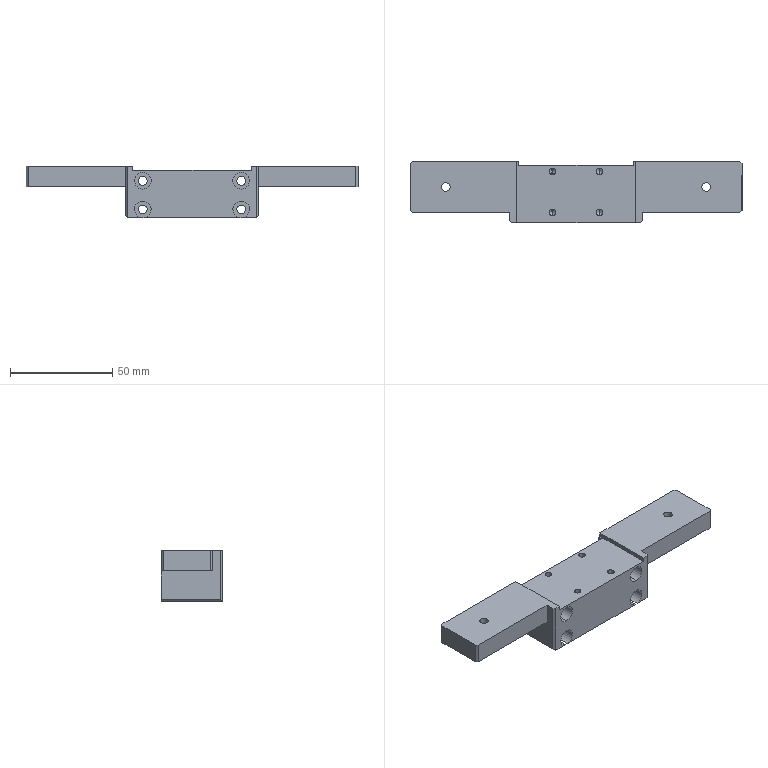Component | SolidWorks | 2018SOLIDWORKS1400000005-1 | 1 solid | 68 faces | box 162 x 30 x 25 mm | volume 60980 mm3 | plane 32 | cylinder 28 | cone 8 | commonest cylinder face diameters 3.3 x8 8.1 x8 4.3 x8 4.2 x4 | material 6061 Alloy
build123d program:
from build123d import *

# Parameters (mm, degrees)
SKETCH1_W                                            = 30
SKETCH1_H                                            = 162
BOSS_EXTRUDE1_DEPTH                                  = 25
SKETCH3_W                                            = 30
SKETCH3_H                                            = 58
CUT_EXTRUDE2_DEPTH                                   = 2
SKETCH4_W                                            = 25
SKETCH4_H                                            = 56
CUT_EXTRUDE3_DEPTH                                   = 2
SKETCH5_W                                            = 15
SKETCH5_H                                            = 48.5
CUT_EXTRUDE4_DEPTH                                   = 90.922
SKETCH7_W                                            = 5
SKETCH7_H                                            = 48.5
CUT_EXTRUDE6_DEPTH                                   = 84.732
HOLE_SIZE_ACCORDING_TO_THE_TYPE_OF_HEX_S_D           = 4.3
HOLE_SIZE_ACCORDING_TO_THE_TYPE_OF_HEX_S_CBORE_D     = 8.1
HOLE_SIZE_ACCORDING_TO_THE_TYPE_OF_HEX_S_CBORE_DEPTH = 24
M4_TAPPED_HOLE1_D                                    = 3.3
M4_TAPPED_HOLE1_DEPTH                                = 12.4
M4_TAPPED_HOLE1_TIP                                  = 0.9914
CHAMFER1_SIZE                                        = 1
M5_TAPPED_HOLE1_D                                    = 4.2
M5_TAPPED_HOLE1_DEPTH                                = 12.4
M5_TAPPED_HOLE1_TIP                                  = 1.262


with BuildPart() as part:
    # Sketch1 → Boss-Extrude1 (new body)
    with BuildSketch(Plane.XY):
        Rectangle(SKETCH1_W, SKETCH1_H)
    extrude(amount=BOSS_EXTRUDE1_DEPTH)

    # Sketch3 → Cut-Extrude2 (cut)
    with BuildSketch(Plane.XY.offset(25)):
        Rectangle(SKETCH3_W, SKETCH3_H)
    extrude(amount=-CUT_EXTRUDE2_DEPTH, mode=Mode.SUBTRACT)

    # Sketch4 → Cut-Extrude3 (cut)
    with BuildSketch(Plane.ZY.offset(-15)):
        with Locations((12.5, 0)):
            Rectangle(SKETCH4_W, SKETCH4_H)
    extrude(amount=CUT_EXTRUDE3_DEPTH, mode=Mode.SUBTRACT)

    # Sketch5 → Cut-Extrude4 (cut, through all)
    with BuildSketch(Plane.ZY.offset(15)):
        with Locations((7.5, 56.75)):
            Rectangle(SKETCH5_W, SKETCH5_H)
        with Locations((7.5, -56.75)):
            Rectangle(SKETCH5_W, SKETCH5_H)
    extrude(amount=-CUT_EXTRUDE4_DEPTH, mode=Mode.SUBTRACT)

    # Sketch7 → Cut-Extrude6 (cut, through all)
    with BuildSketch(Plane(origin=(0, 0, 15), x_dir=(-1, 0, 0), z_dir=(0, 0, -1))):
        with Locations((12.5, 56.75)):
            Rectangle(SKETCH7_W, SKETCH7_H)
        with Locations((12.5, -56.75)):
            Rectangle(SKETCH7_W, SKETCH7_H)
    extrude(amount=-CUT_EXTRUDE6_DEPTH, mode=Mode.SUBTRACT)

    # Hole Size according to the type of hex s (through all)
    with Locations(Plane.ZY.offset(15)):
        with Locations((4, 24), (18, 24), (4, -24), (18, -24)):
            CounterBoreHole(HOLE_SIZE_ACCORDING_TO_THE_TYPE_OF_HEX_S_D / 2, HOLE_SIZE_ACCORDING_TO_THE_TYPE_OF_HEX_S_CBORE_D / 2, HOLE_SIZE_ACCORDING_TO_THE_TYPE_OF_HEX_S_CBORE_DEPTH)

    # M4 Tapped Hole1
    with Locations(Plane.XY.offset(23)):
        with Locations((-10, 11.5), (10, 11.5), (10, -11.5), (-10, -11.5)):
            Hole(M4_TAPPED_HOLE1_D / 2, depth=M4_TAPPED_HOLE1_DEPTH)
            with Locations((0, 0, -(M4_TAPPED_HOLE1_DEPTH + M4_TAPPED_HOLE1_TIP / 2))):  # 118° drill point
                Cone(0, M4_TAPPED_HOLE1_D / 2, M4_TAPPED_HOLE1_TIP, mode=Mode.SUBTRACT)

    # Chamfer1
    chamfer1_edges = [part.edges().sort_by_distance(p)[0] for p in [
        (0, 32.5, 0),
        (-15, 32.5, 12.5),
        (0, -32.5, 0),
        (-15, -32.5, 12.5),
        (15, -81, 20),
        (15, 81, 20),
        (-10, 81, 20),
        (-10, -81, 20),
    ]]
    chamfer(chamfer1_edges, length=CHAMFER1_SIZE)

    # M5 Tapped Hole1
    with Locations(Plane.XY.offset(25)):
        with Locations((2.5, -63.5), (2.5, 63.5)):
            Hole(M5_TAPPED_HOLE1_D / 2, depth=M5_TAPPED_HOLE1_DEPTH)
            with Locations((0, 0, -(M5_TAPPED_HOLE1_DEPTH + M5_TAPPED_HOLE1_TIP / 2))):  # 118° drill point
                Cone(0, M5_TAPPED_HOLE1_D / 2, M5_TAPPED_HOLE1_TIP, mode=Mode.SUBTRACT)


solid = part.part

# Placed as in the assembly
solid = solid.moved(Location((163.212, -57.5, 186), (0, 0, 90)))